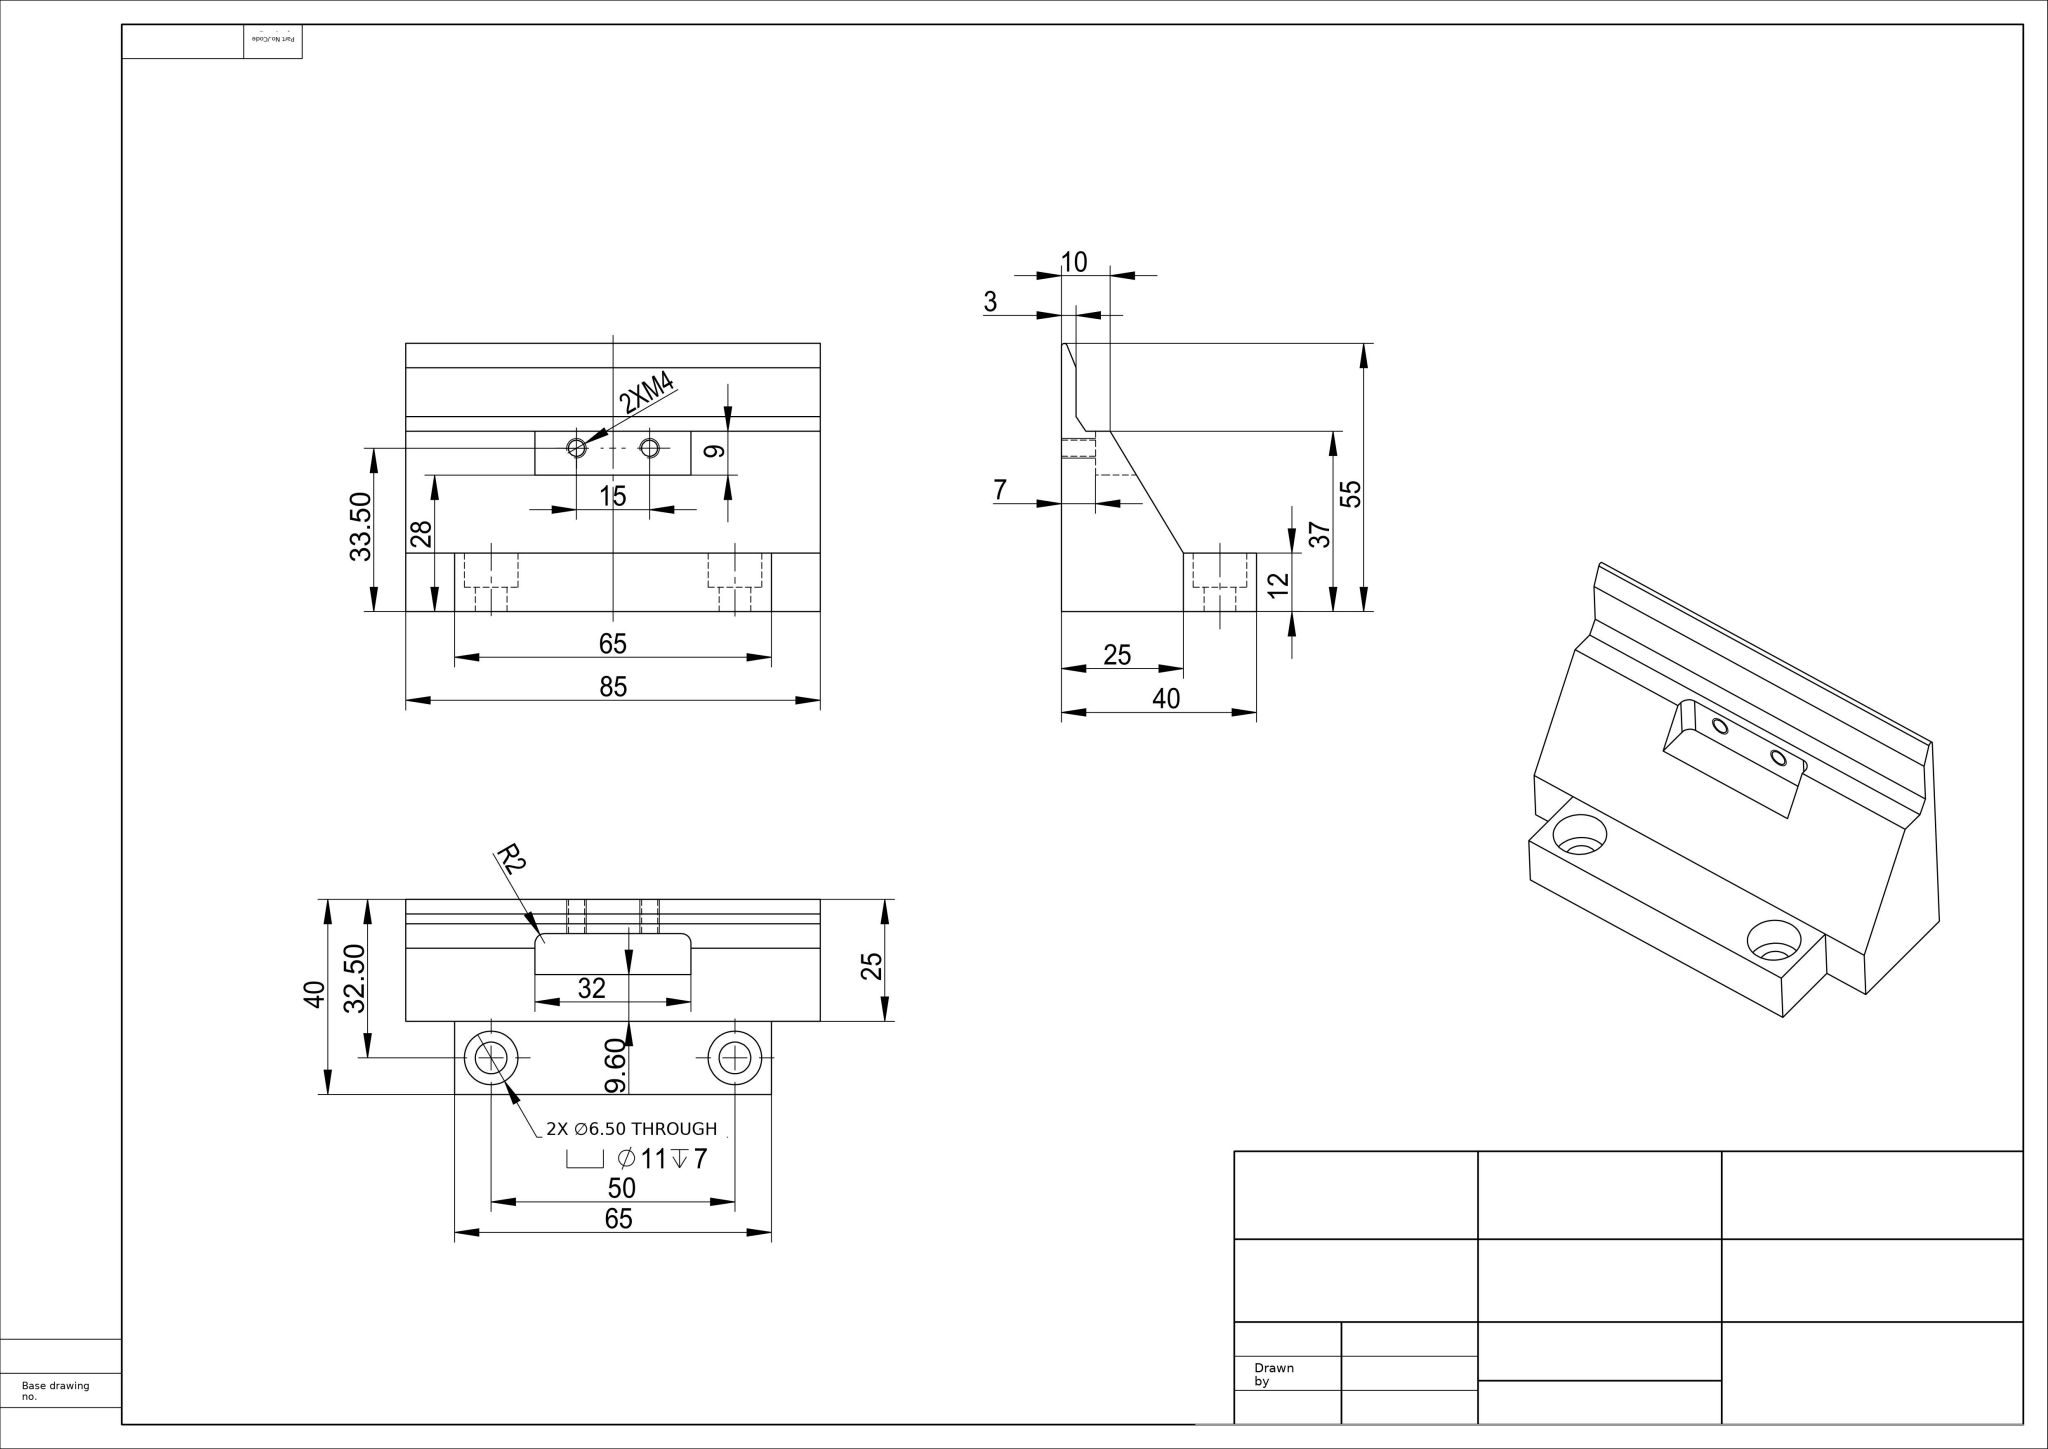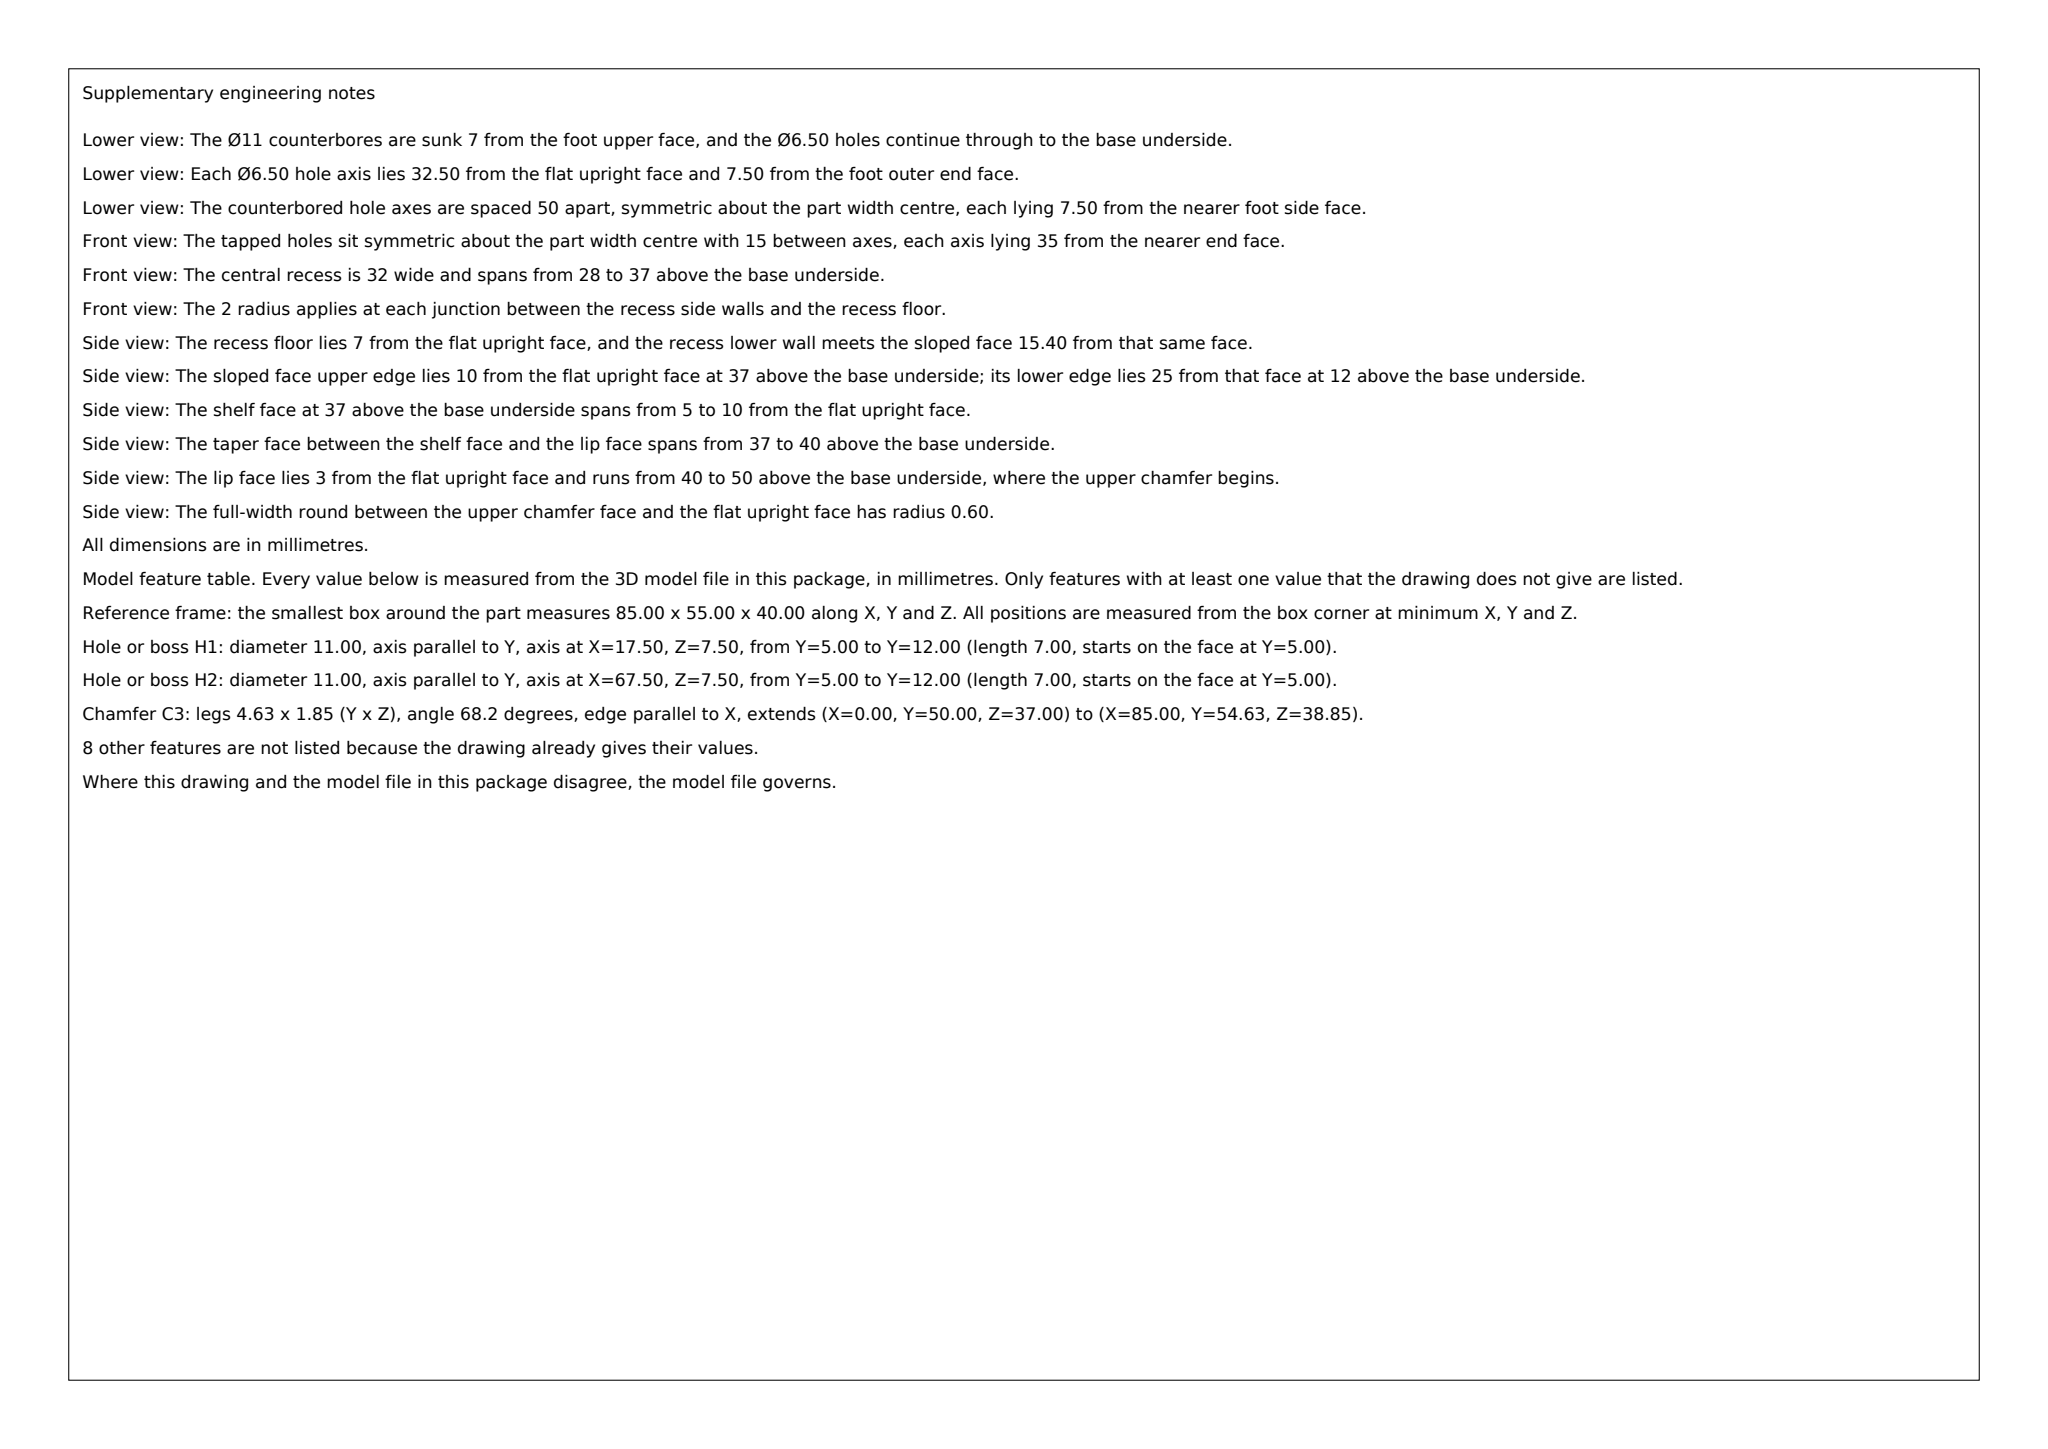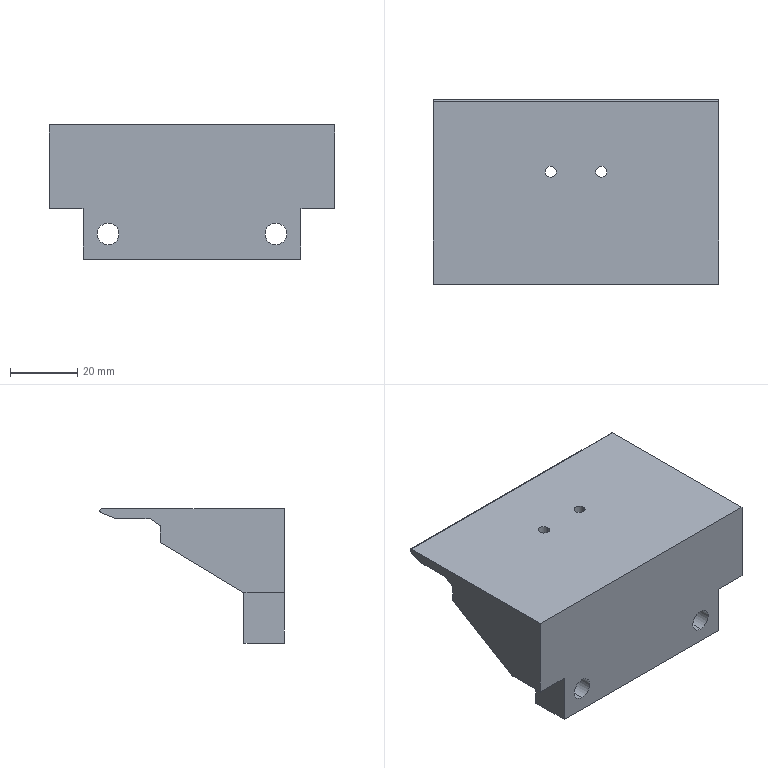Part | SolidWorks | mm | 1 solid | 36 faces | box 85 x 55 x 40 mm | volume 75390 mm3 | plane 21 | cylinder 15 | commonest cylinder face diameters 3.3 x4 11 x4 6.5 x4 4 x2 1.193 x1
Drawing notes:
2X M4 DP 7 THD (Ø3.3 DRILL DP 7) - TAPPED FROM FRONT FACE | from the solid: cylinders dia 3.3 axis z at (35.0,33.5) and (50.0,33.5), length 7.0, blind